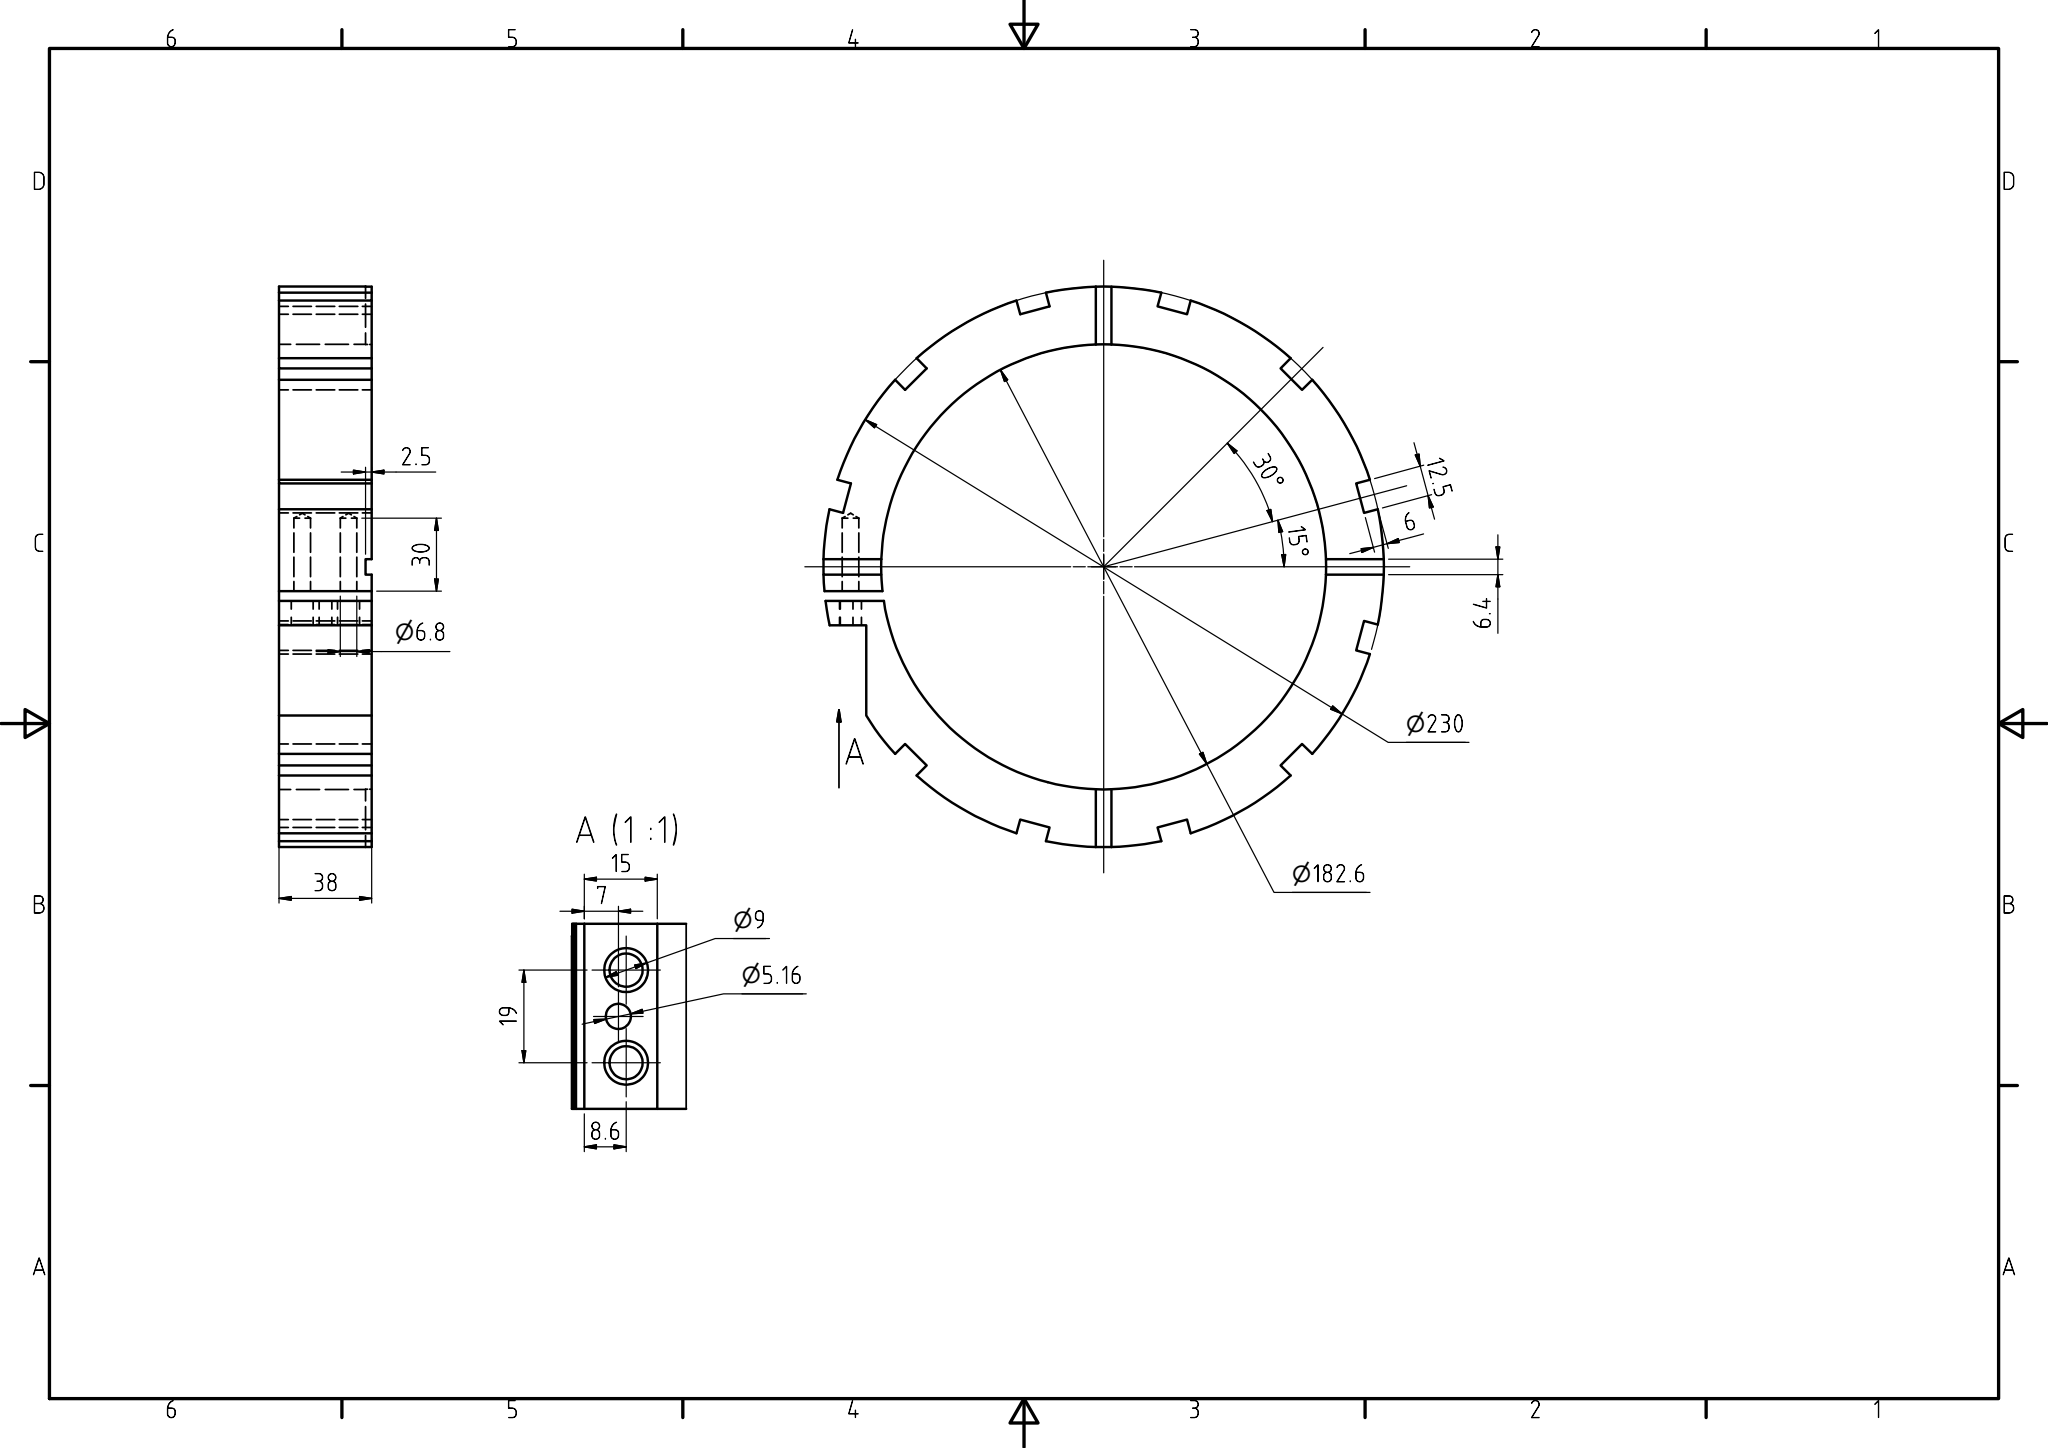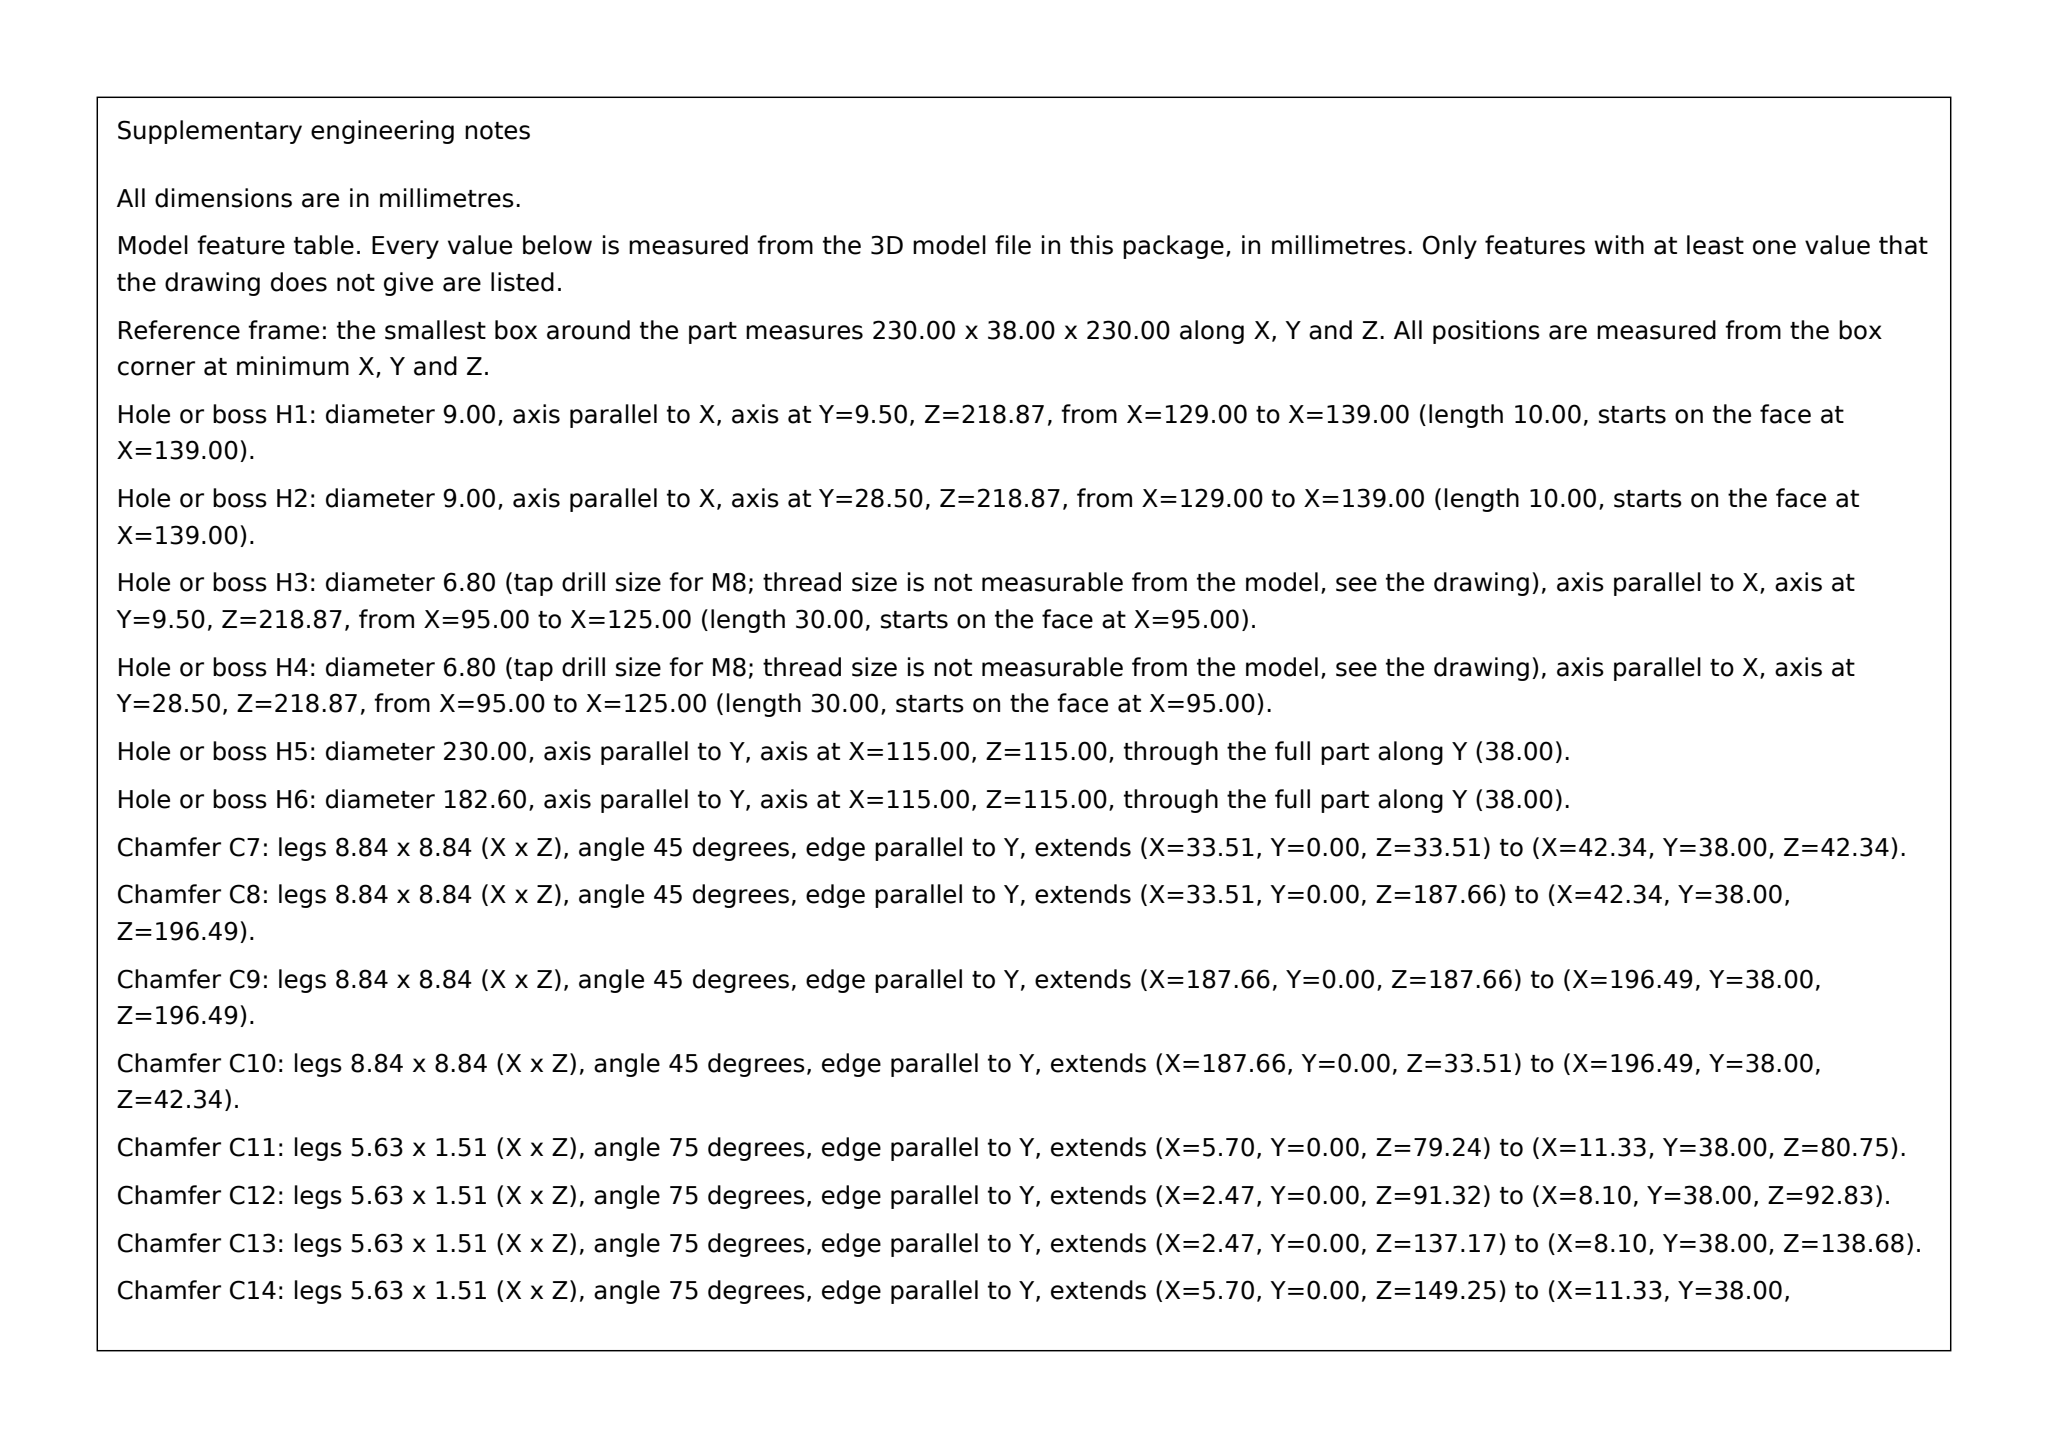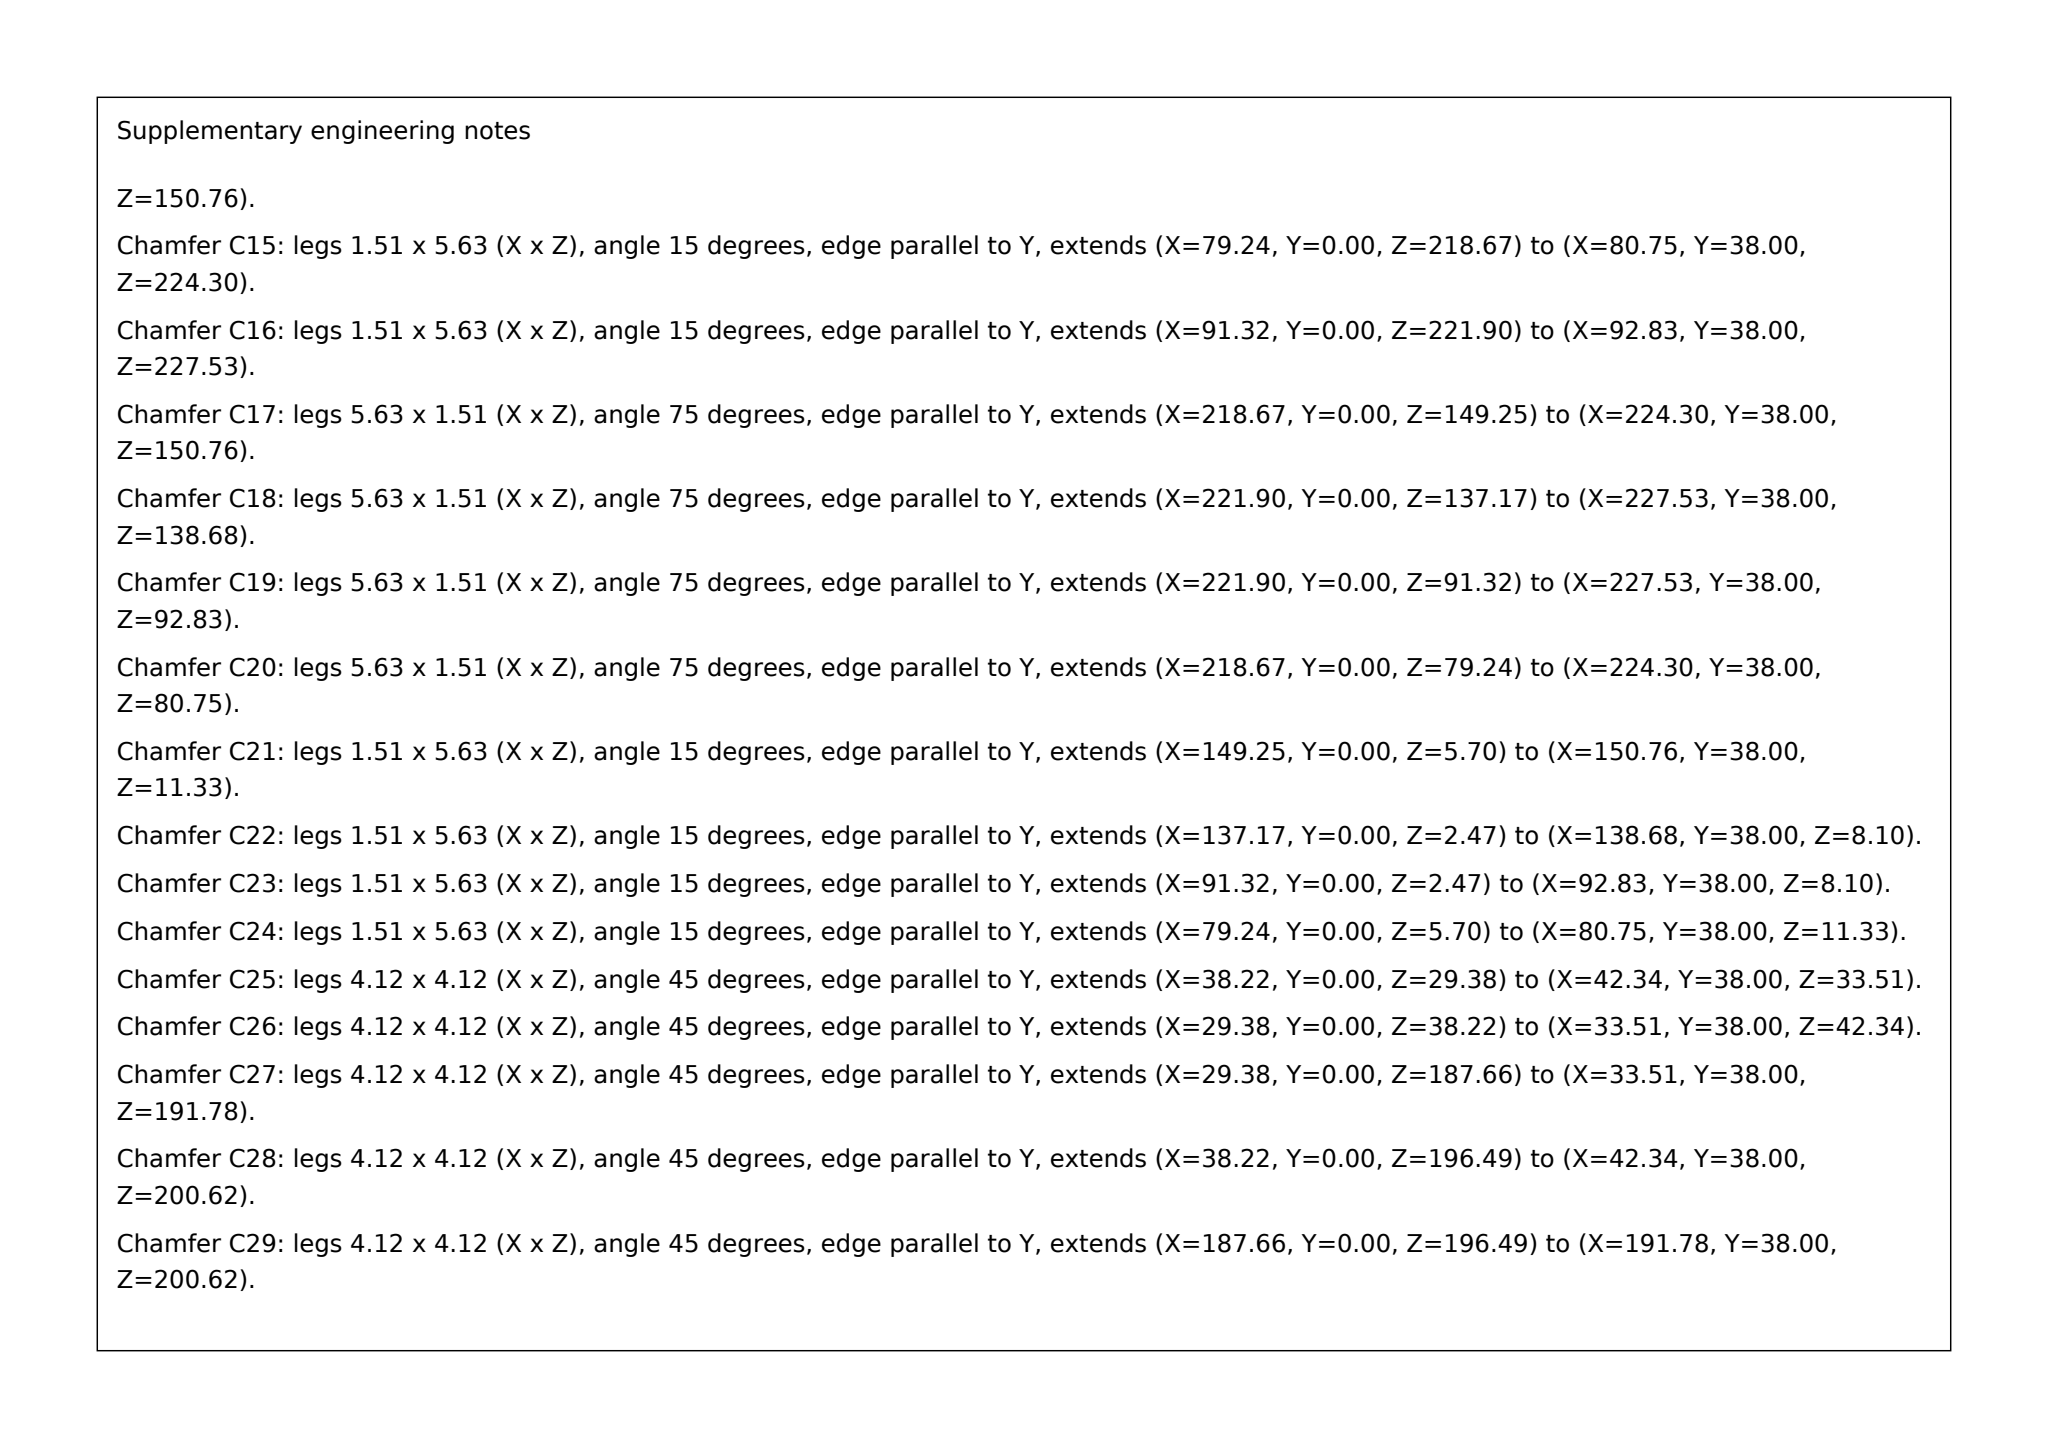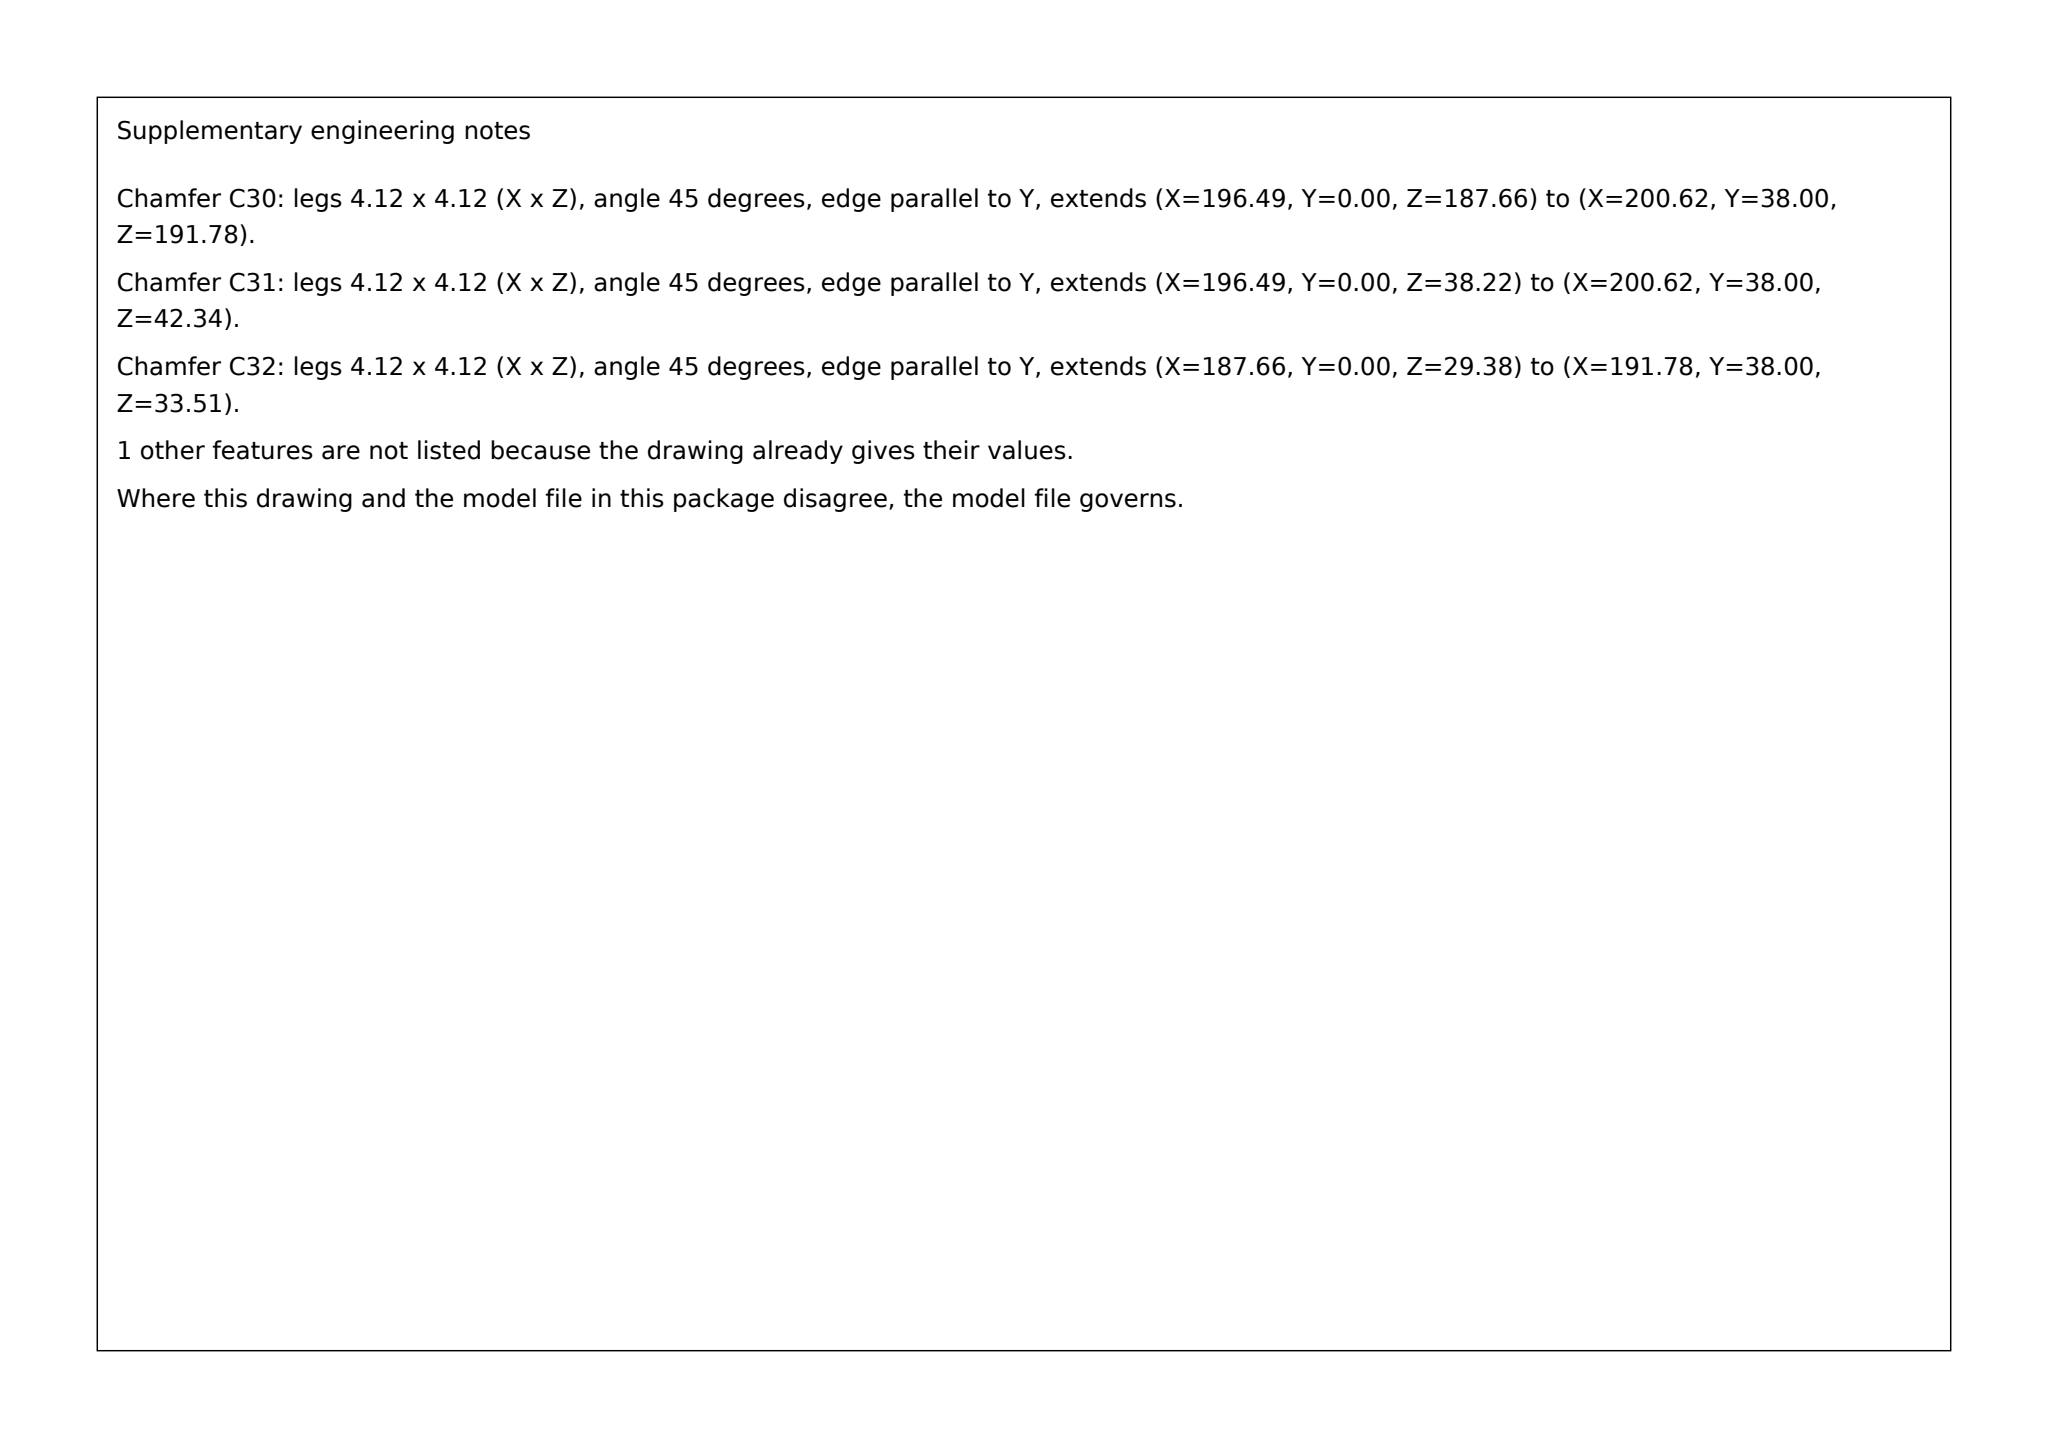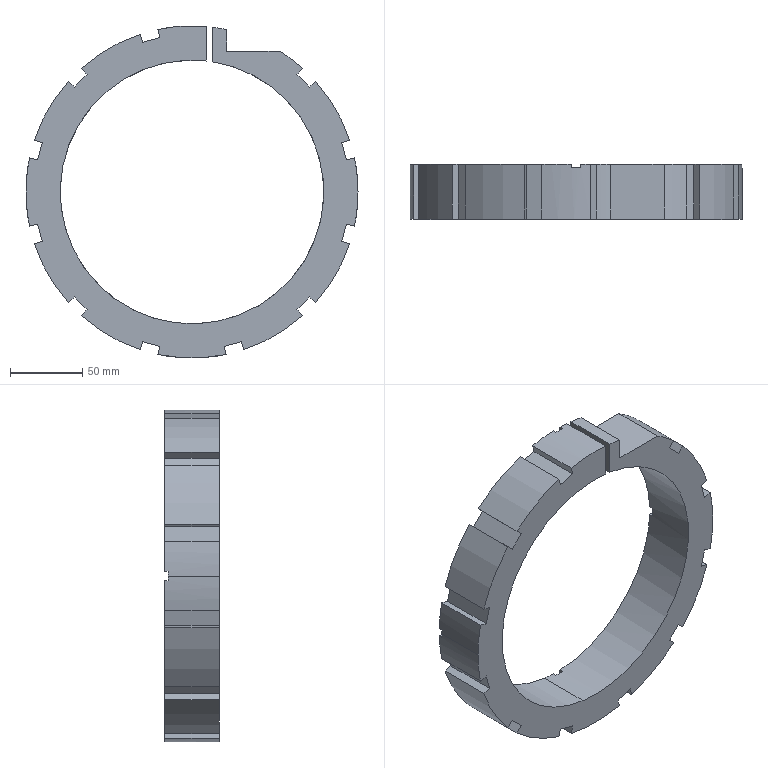Part | SolidWorks | mm | 1 solid | 86 faces | box 230 x 38 x 230 mm | volume 531453 mm3 | plane 55 | cylinder 27 | cone 4 | commonest cylinder face diameters 230 x15 9 x4 6.8 x4 182.6 x2 5.16 x2